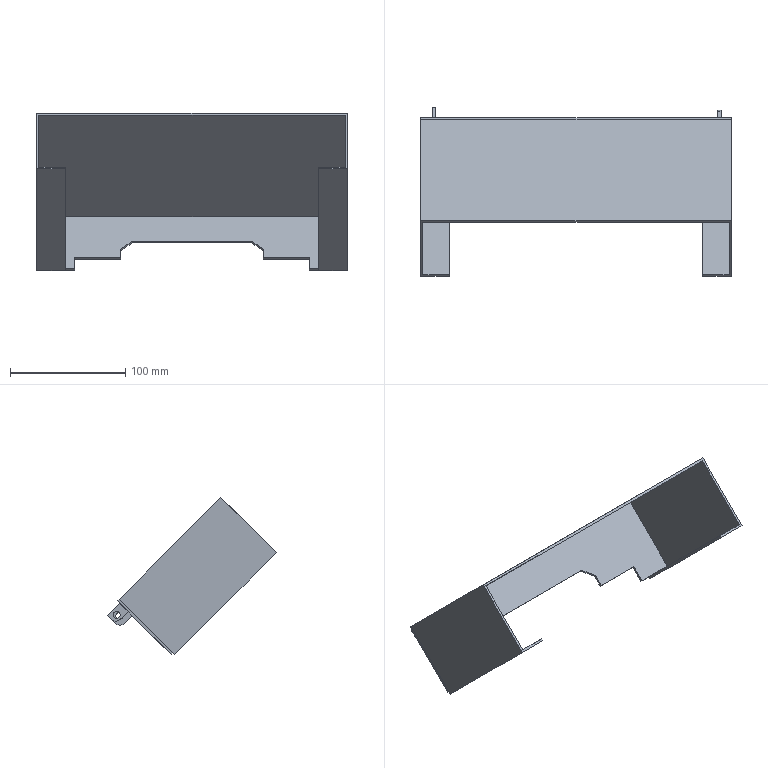Component | SolidWorks | Section1-1 | 2 solids | 47 faces | box 270 x 146.37 x 136.47 mm | volume 138075 mm3 | plane 40 | cylinder 7 | commonest cylinder face diameters 6 x4 10 x3
build123d program:
from build123d import *

# Parameters (mm, degrees)
EXTRUDE_THIN1_DEPTH = 125
BOSS_EXTRUDE3_DEPTH = 2
SKETCH4_W           = 3
SKETCH4_H           = 15
SKETCH4_H_2         = 10
BOSS_EXTRUDE4_DEPTH = 15
FILLET1_R           = 5
FILLET2_R           = 5
SKETCH5_R           = 3
CUT_EXTRUDE1_DEPTH  = 3
SKETCH6_R           = 3
CUT_EXTRUDE2_DEPTH  = 3


with BuildPart() as part:
    # Sketch1 → Extrude-Thin1 (new body)
    with BuildSketch(Plane.XY):
        Polygon((-32.5, -61), (-57.5, -61), (-57.5, 7), (212.5, 7), (212.5, -61), (187.5, -61), (187.5, -59), (210.5, -59), (210.5, 5), (-55.5, 5), (-55.5, -59), (-32.5, -59), align=None)
    extrude(amount=EXTRUDE_THIN1_DEPTH)


with BuildPart() as body_2:
    # Sketch3 → Boss-Extrude3 (new body)
    with BuildSketch(Plane(origin=(0, 0, 0), x_dir=(-1, 0, 0), z_dir=(0, 0, -1))):
        Polygon((-212.5, -59), (-212.5, 7), (57.5, 7), (57.5, -59), (24.5, -59), (24.5, -55.817), (24.5, -45), (-15.5, -45), (-15.5, -35), (-25.5, -25), (-129.5, -25), (-139.5, -35), (-139.5, -45), (-179.5, -45), (-179.5, -59), align=None)
    extrude(amount=BOSS_EXTRUDE3_DEPTH)

    # Sketch4 → Boss-Extrude4 (add)
    with BuildSketch(Plane(origin=(0, 0, -2), x_dir=(-1, 0, 0), z_dir=(0, 0, -1))):
        with Locations((-202, -3.5)):
            Rectangle(SKETCH4_W, SKETCH4_H)
        with Locations((46, -0.9998)):
            Rectangle(SKETCH4_W, SKETCH4_H_2)
    extrude(amount=BOSS_EXTRUDE4_DEPTH)

    # Fillet1
    fillet1_edges = [body_2.edges().sort_by_distance(p)[0] for p in [
        (-46, -6, -17),
    ]]
    fillet(fillet1_edges, radius=FILLET1_R)

    # Fillet2
    fillet2_edges = [body_2.edges().sort_by_distance(p)[0] for p in [
        (202, -11, -17),
        (202, 4, -17),
    ]]
    fillet(fillet2_edges, radius=FILLET2_R)

    # Sketch5 → Cut-Extrude1 (cut)
    with BuildSketch(Plane(origin=(203.5, 0, 0), x_dir=(0, 0, -1), z_dir=(1, 0, 0))):
        with Locations((10.225, -3.5)):
            Circle(SKETCH5_R)
    extrude(amount=-CUT_EXTRUDE1_DEPTH, mode=Mode.SUBTRACT)

    # Sketch6 → Cut-Extrude2 (cut)
    with BuildSketch(Plane.ZY.offset(47.5)):
        with Locations((-11.103, -0.9998)):
            Circle(SKETCH6_R)
    extrude(amount=-CUT_EXTRUDE2_DEPTH, mode=Mode.SUBTRACT)


solid = Compound([part.part, body_2.part])

# Placed as in the assembly
solid = solid.moved(Location((41.324, -143.201, -32.779), (45, 0, 0)))